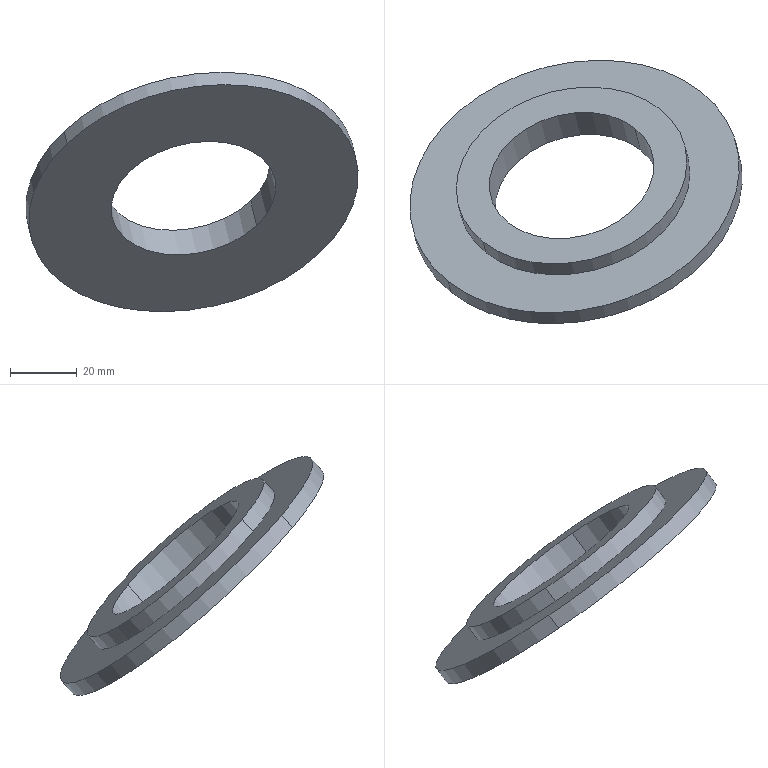Component | SolidWorks | FrictionWasher2-1 | 1 solid | 9 faces | box 99.33 x 78.81 x 71.5 mm | volume 38877 mm3 | cylinder 6 | plane 3 | commonest cylinder face diameters 70 x2 50 x2 100 x2 | material Copper
build123d program:
from build123d import *

# Parameters (mm, degrees)
SKETCH1_R           = 50
SKETCH1_R_2         = 35
BOSS_EXTRUDE1_DEPTH = 5
SKETCH1_3_R         = 35
SKETCH1_3_R_2       = 25
BOSS_EXTRUDE2_DEPTH = 10


with BuildPart() as part:
    # Sketch1 → Boss-Extrude1 (new body)
    with BuildSketch(Plane(origin=(0, 0, 0), x_dir=(1, 0, 0), z_dir=(0, 1, 0))):
        with Locations(Location((0, 0, 0), (0, 0, 270))):
            Circle(SKETCH1_R)
        with Locations(Location((0, 0, 0), (0, 0, 270))):
            Circle(SKETCH1_R_2, mode=Mode.SUBTRACT)
    extrude(amount=BOSS_EXTRUDE1_DEPTH)

    # Sketch1_3 → Boss-Extrude2 (add)
    with BuildSketch(Plane(origin=(0, 0, 0), x_dir=(1, 0, 0), z_dir=(0, 1, 0))):
        with Locations(Location((0, 0, 0), (0, 0, 270))):
            Circle(SKETCH1_3_R)
        with Locations(Location((0, 0, 0), (0, 0, 270))):
            Circle(SKETCH1_3_R_2, mode=Mode.SUBTRACT)
    extrude(amount=BOSS_EXTRUDE2_DEPTH)


solid = part.part

# Placed as in the assembly
solid = solid.moved(Location((-353.935, -1548.439, -88.002), (173.543, -77.716, 124.647)))
STEP:
#1=COLOUR_RGB('',0.7922,0.8196,0.9333);
#2=FILL_AREA_STYLE_COLOUR('',#1);
#3=FILL_AREA_STYLE('',(#2));
#4=SURFACE_STYLE_FILL_AREA(#3);
#5=SURFACE_SIDE_STYLE('',(#4));
#6=SURFACE_STYLE_USAGE(.BOTH.,#5);
#7=PRESENTATION_STYLE_ASSIGNMENT((#6));
#8=CARTESIAN_POINT('',(-12.963,-59.921,-3.626));
#9=VERTEX_POINT('',#8);
#10=CARTESIAN_POINT('',(-15.044,-61.487,-2.725));
#11=VERTEX_POINT('',#10);
#12=CARTESIAN_POINT('',(-14.003,-60.704,-3.175));
#13=DIRECTION('',(-0.175,0.6553,0.7348));
#14=DIRECTION('',(0.755,0.5683,-0.327));
#15=AXIS2_PLACEMENT_3D('',#12,#13,#14);
#16=CIRCLE('',#15,1.378);
#17=EDGE_CURVE('',#9,#11,#16,.T.);
#18=ORIENTED_EDGE('',*,*,#17,.F.);
#19=CARTESIAN_POINT('',(-12.928,-60.05,-3.771));
#20=VERTEX_POINT('',#19);
#21=CARTESIAN_POINT('',(-12.963,-59.921,-3.626));
#22=DIRECTION('',(0.175,-0.6553,-0.7348));
#23=VECTOR('',#22,39.37);
#24=LINE('',#21,#23);
#25=EDGE_CURVE('',#9,#20,#24,.T.);
#26=ORIENTED_EDGE('',*,*,#25,.T.);
#27=CARTESIAN_POINT('',(-15.009,-61.616,-2.869));
#28=VERTEX_POINT('',#27);
#29=CARTESIAN_POINT('',(-13.969,-60.833,-3.32));
#30=DIRECTION('',(-0.175,0.6553,0.7348));
#31=DIRECTION('',(0.755,0.5683,-0.327));
#32=AXIS2_PLACEMENT_3D('',#29,#30,#31);
#33=CIRCLE('',#32,1.378);
#34=EDGE_CURVE('',#20,#28,#33,.T.);
#35=ORIENTED_EDGE('',*,*,#34,.T.);
#36=CARTESIAN_POINT('',(-15.044,-61.487,-2.725));
#37=DIRECTION('',(0.175,-0.6553,-0.7348));
#38=VECTOR('',#37,39.37);
#39=LINE('',#36,#38);
#40=EDGE_CURVE('',#11,#28,#39,.T.);
#41=ORIENTED_EDGE('',*,*,#40,.F.);
#42=EDGE_LOOP('',(#18,#26,#35,#41));
#43=FACE_OUTER_BOUND('',#42,.T.);
#44=CARTESIAN_POINT('',(-14.003,-60.704,-3.175));
#45=DIRECTION('',(0.175,-0.6553,-0.7348));
#46=DIRECTION('',(-0.755,-0.5683,0.327));
#47=AXIS2_PLACEMENT_3D('',#44,#45,#46);
#48=CYLINDRICAL_SURFACE('',#47,1.378);
#49=ADVANCED_FACE('',(#43),#48,.T.);
#50=CARTESIAN_POINT('',(-14.747,-61.264,-2.854));
#51=VERTEX_POINT('',#50);
#52=CARTESIAN_POINT('',(-13.26,-60.145,-3.497));
#53=VERTEX_POINT('',#52);
#54=CARTESIAN_POINT('',(-14.003,-60.704,-3.175));
#55=DIRECTION('',(-0.175,0.6553,0.7348));
#56=DIRECTION('',(0.755,0.5683,-0.327));
#57=AXIS2_PLACEMENT_3D('',#54,#55,#56);
#58=CIRCLE('',#57,0.9843);
#59=EDGE_CURVE('',#51,#53,#58,.T.);
#60=ORIENTED_EDGE('',*,*,#59,.T.);
#61=CARTESIAN_POINT('',(-13.191,-60.403,-3.786));
#62=VERTEX_POINT('',#61);
#63=CARTESIAN_POINT('',(-13.26,-60.145,-3.497));
#64=DIRECTION('',(0.175,-0.6553,-0.7348));
#65=VECTOR('',#64,39.37);
#66=LINE('',#63,#65);
#67=EDGE_CURVE('',#53,#62,#66,.T.);
#68=ORIENTED_EDGE('',*,*,#67,.T.);
#69=CARTESIAN_POINT('',(-14.678,-61.522,-3.143));
#70=VERTEX_POINT('',#69);
#71=CARTESIAN_POINT('',(-13.934,-60.962,-3.465));
#72=DIRECTION('',(-0.175,0.6553,0.7348));
#73=DIRECTION('',(0.755,0.5683,-0.327));
#74=AXIS2_PLACEMENT_3D('',#71,#72,#73);
#75=CIRCLE('',#74,0.9843);
#76=EDGE_CURVE('',#70,#62,#75,.T.);
#77=ORIENTED_EDGE('',*,*,#76,.F.);
#78=CARTESIAN_POINT('',(-14.747,-61.264,-2.854));
#79=DIRECTION('',(0.175,-0.6553,-0.7348));
#80=VECTOR('',#79,39.37);
#81=LINE('',#78,#80);
#82=EDGE_CURVE('',#51,#70,#81,.T.);
#83=ORIENTED_EDGE('',*,*,#82,.F.);
#84=EDGE_LOOP('',(#60,#68,#77,#83));
#85=FACE_OUTER_BOUND('',#84,.T.);
#86=CARTESIAN_POINT('',(-14.003,-60.704,-3.175));
#87=DIRECTION('',(0.175,-0.6553,-0.7348));
#88=DIRECTION('',(-0.755,-0.5683,0.327));
#89=AXIS2_PLACEMENT_3D('',#86,#87,#88);
#90=CYLINDRICAL_SURFACE('',#89,0.9843);
#91=ADVANCED_FACE('',(#85),#90,.F.);
#92=CARTESIAN_POINT('',(-12.483,-59.714,-3.964));
#93=VERTEX_POINT('',#92);
#94=CARTESIAN_POINT('',(-15.455,-61.952,-2.676));
#95=VERTEX_POINT('',#94);
#96=CARTESIAN_POINT('',(-13.969,-60.833,-3.32));
#97=DIRECTION('',(-0.175,0.6553,0.7348));
#98=DIRECTION('',(0.755,0.5683,-0.327));
#99=AXIS2_PLACEMENT_3D('',#96,#97,#98);
#100=CIRCLE('',#99,1.969);
#101=EDGE_CURVE('',#93,#95,#100,.T.);
#102=ORIENTED_EDGE('',*,*,#101,.F.);
#103=CARTESIAN_POINT('',(-12.448,-59.843,-4.108));
#104=VERTEX_POINT('',#103);
#105=CARTESIAN_POINT('',(-12.483,-59.714,-3.964));
#106=DIRECTION('',(0.175,-0.6553,-0.7348));
#107=VECTOR('',#106,39.37);
#108=LINE('',#105,#107);
#109=EDGE_CURVE('',#93,#104,#108,.T.);
#110=ORIENTED_EDGE('',*,*,#109,.T.);
#111=CARTESIAN_POINT('',(-15.421,-62.081,-2.821));
#112=VERTEX_POINT('',#111);
#113=CARTESIAN_POINT('',(-13.934,-60.962,-3.465));
#114=DIRECTION('',(-0.175,0.6553,0.7348));
#115=DIRECTION('',(0.755,0.5683,-0.327));
#116=AXIS2_PLACEMENT_3D('',#113,#114,#115);
#117=CIRCLE('',#116,1.969);
#118=EDGE_CURVE('',#104,#112,#117,.T.);
#119=ORIENTED_EDGE('',*,*,#118,.T.);
#120=CARTESIAN_POINT('',(-15.455,-61.952,-2.676));
#121=DIRECTION('',(0.175,-0.6553,-0.7348));
#122=VECTOR('',#121,39.37);
#123=LINE('',#120,#122);
#124=EDGE_CURVE('',#95,#112,#123,.T.);
#125=ORIENTED_EDGE('',*,*,#124,.F.);
#126=EDGE_LOOP('',(#102,#110,#119,#125));
#127=FACE_OUTER_BOUND('',#126,.T.);
#128=CARTESIAN_POINT('',(-13.969,-60.833,-3.32));
#129=DIRECTION('',(0.175,-0.6553,-0.7348));
#130=DIRECTION('',(-0.755,-0.5683,0.327));
#131=AXIS2_PLACEMENT_3D('',#128,#129,#130);
#132=CYLINDRICAL_SURFACE('',#131,1.969);
#133=ADVANCED_FACE('',(#127),#132,.T.);
#134=ORIENTED_EDGE('',*,*,#109,.F.);
#135=CARTESIAN_POINT('',(-13.969,-60.833,-3.32));
#136=DIRECTION('',(-0.175,0.6553,0.7348));
#137=DIRECTION('',(0.755,0.5683,-0.327));
#138=AXIS2_PLACEMENT_3D('',#135,#136,#137);
#139=CIRCLE('',#138,1.969);
#140=EDGE_CURVE('',#95,#93,#139,.T.);
#141=ORIENTED_EDGE('',*,*,#140,.F.);
#142=ORIENTED_EDGE('',*,*,#124,.T.);
#143=CARTESIAN_POINT('',(-13.934,-60.962,-3.465));
#144=DIRECTION('',(-0.175,0.6553,0.7348));
#145=DIRECTION('',(0.755,0.5683,-0.327));
#146=AXIS2_PLACEMENT_3D('',#143,#144,#145);
#147=CIRCLE('',#146,1.969);
#148=EDGE_CURVE('',#112,#104,#147,.T.);
#149=ORIENTED_EDGE('',*,*,#148,.T.);
#150=EDGE_LOOP('',(#134,#141,#142,#149));
#151=FACE_OUTER_BOUND('',#150,.T.);
#152=CARTESIAN_POINT('',(-13.969,-60.833,-3.32));
#153=DIRECTION('',(0.175,-0.6553,-0.7348));
#154=DIRECTION('',(-0.755,-0.5683,0.327));
#155=AXIS2_PLACEMENT_3D('',#152,#153,#154);
#156=CYLINDRICAL_SURFACE('',#155,1.969);
#157=ADVANCED_FACE('',(#151),#156,.T.);
#158=CARTESIAN_POINT('',(-13.969,-60.833,-3.32));
#159=DIRECTION('',(-0.175,0.6553,0.7348));
#160=DIRECTION('',(0.755,0.5683,-0.327));
#161=AXIS2_PLACEMENT_3D('',#158,#159,#160);
#162=CIRCLE('',#161,1.378);
#163=EDGE_CURVE('',#28,#20,#162,.T.);
#164=ORIENTED_EDGE('',*,*,#163,.F.);
#165=ORIENTED_EDGE('',*,*,#34,.F.);
#166=EDGE_LOOP('',(#164,#165));
#167=FACE_BOUND('',#166,.T.);
#168=ORIENTED_EDGE('',*,*,#140,.T.);
#169=ORIENTED_EDGE('',*,*,#101,.T.);
#170=EDGE_LOOP('',(#168,#169));
#171=FACE_OUTER_BOUND('',#170,.T.);
#172=CARTESIAN_POINT('',(-13.969,-60.833,-3.32));
#173=DIRECTION('',(-0.175,0.6553,0.7348));
#174=DIRECTION('',(0.755,0.5683,-0.327));
#175=AXIS2_PLACEMENT_3D('',#172,#173,#174);
#176=PLANE('',#175);
#177=ADVANCED_FACE('',(#167,#171),#176,.T.);
#178=ORIENTED_EDGE('',*,*,#148,.F.);
#179=ORIENTED_EDGE('',*,*,#118,.F.);
#180=EDGE_LOOP('',(#178,#179));
#181=FACE_OUTER_BOUND('',#180,.T.);
#182=ORIENTED_EDGE('',*,*,#76,.T.);
#183=CARTESIAN_POINT('',(-13.934,-60.962,-3.465));
#184=DIRECTION('',(-0.175,0.6553,0.7348));
#185=DIRECTION('',(0.755,0.5683,-0.327));
#186=AXIS2_PLACEMENT_3D('',#183,#184,#185);
#187=CIRCLE('',#186,0.9843);
#188=EDGE_CURVE('',#62,#70,#187,.T.);
#189=ORIENTED_EDGE('',*,*,#188,.T.);
#190=EDGE_LOOP('',(#182,#189));
#191=FACE_BOUND('',#190,.T.);
#192=CARTESIAN_POINT('',(-13.934,-60.962,-3.465));
#193=DIRECTION('',(-0.175,0.6553,0.7348));
#194=DIRECTION('',(0.755,0.5683,-0.327));
#195=AXIS2_PLACEMENT_3D('',#192,#193,#194);
#196=PLANE('',#195);
#197=ADVANCED_FACE('',(#181,#191),#196,.F.);
#198=ORIENTED_EDGE('',*,*,#67,.F.);
#199=CARTESIAN_POINT('',(-14.003,-60.704,-3.175));
#200=DIRECTION('',(-0.175,0.6553,0.7348));
#201=DIRECTION('',(0.755,0.5683,-0.327));
#202=AXIS2_PLACEMENT_3D('',#199,#200,#201);
#203=CIRCLE('',#202,0.9843);
#204=EDGE_CURVE('',#53,#51,#203,.T.);
#205=ORIENTED_EDGE('',*,*,#204,.T.);
#206=ORIENTED_EDGE('',*,*,#82,.T.);
#207=ORIENTED_EDGE('',*,*,#188,.F.);
#208=EDGE_LOOP('',(#198,#205,#206,#207));
#209=FACE_OUTER_BOUND('',#208,.T.);
#210=CARTESIAN_POINT('',(-14.003,-60.704,-3.175));
#211=DIRECTION('',(0.175,-0.6553,-0.7348));
#212=DIRECTION('',(-0.755,-0.5683,0.327));
#213=AXIS2_PLACEMENT_3D('',#210,#211,#212);
#214=CYLINDRICAL_SURFACE('',#213,0.9843);
#215=ADVANCED_FACE('',(#209),#214,.F.);
#216=ORIENTED_EDGE('',*,*,#25,.F.);
#217=CARTESIAN_POINT('',(-14.003,-60.704,-3.175));
#218=DIRECTION('',(-0.175,0.6553,0.7348));
#219=DIRECTION('',(0.755,0.5683,-0.327));
#220=AXIS2_PLACEMENT_3D('',#217,#218,#219);
#221=CIRCLE('',#220,1.378);
#222=EDGE_CURVE('',#11,#9,#221,.T.);
#223=ORIENTED_EDGE('',*,*,#222,.F.);
#224=ORIENTED_EDGE('',*,*,#40,.T.);
#225=ORIENTED_EDGE('',*,*,#163,.T.);
#226=EDGE_LOOP('',(#216,#223,#224,#225));
#227=FACE_OUTER_BOUND('',#226,.T.);
#228=CARTESIAN_POINT('',(-14.003,-60.704,-3.175));
#229=DIRECTION('',(0.175,-0.6553,-0.7348));
#230=DIRECTION('',(-0.755,-0.5683,0.327));
#231=AXIS2_PLACEMENT_3D('',#228,#229,#230);
#232=CYLINDRICAL_SURFACE('',#231,1.378);
#233=ADVANCED_FACE('',(#227),#232,.T.);
#234=ORIENTED_EDGE('',*,*,#59,.F.);
#235=ORIENTED_EDGE('',*,*,#204,.F.);
#236=EDGE_LOOP('',(#234,#235));
#237=FACE_BOUND('',#236,.T.);
#238=ORIENTED_EDGE('',*,*,#222,.T.);
#239=ORIENTED_EDGE('',*,*,#17,.T.);
#240=EDGE_LOOP('',(#238,#239));
#241=FACE_OUTER_BOUND('',#240,.T.);
#242=CARTESIAN_POINT('',(-14.003,-60.704,-3.175));
#243=DIRECTION('',(-0.175,0.6553,0.7348));
#244=DIRECTION('',(0.755,0.5683,-0.327));
#245=AXIS2_PLACEMENT_3D('',#242,#243,#244);
#246=PLANE('',#245);
#247=ADVANCED_FACE('',(#237,#241),#246,.T.);
#248=CLOSED_SHELL('',(#49,#91,#133,#157,#177,#197,#215,#233,#247));
#249=MANIFOLD_SOLID_BREP('',#248);
#250=STYLED_ITEM('',(#7),#249);
#251=PRESENTATION_LAYER_ASSIGNMENT('','',(#250));
#252=CARTESIAN_POINT('',(0.,0.,0.));
#253=DIRECTION('',(0.,0.,1.));
#254=DIRECTION('',(1.,0.,0.));
#255=AXIS2_PLACEMENT_3D('',#252,#253,#254);
#256=(LENGTH_UNIT()NAMED_UNIT(*)SI_UNIT($,.METRE.));
#257=LENGTH_MEASURE_WITH_UNIT(LENGTH_MEASURE(0.0254),#256);
#258=DIMENSIONAL_EXPONENTS(1.,0.,0.,0.,0.,0.,0.);
#259=(CONVERSION_BASED_UNIT('',#257)LENGTH_UNIT()NAMED_UNIT(#258));
#260=UNCERTAINTY_MEASURE_WITH_UNIT(LENGTH_MEASURE(0.00001),#259,'','');
#261=(NAMED_UNIT(*)PLANE_ANGLE_UNIT()SI_UNIT($,.RADIAN.));
#262=(NAMED_UNIT(*)SI_UNIT($,.STERADIAN.)SOLID_ANGLE_UNIT());
#263=(GEOMETRIC_REPRESENTATION_CONTEXT(3)GLOBAL_UNCERTAINTY_ASSIGNED_CONTEXT((#260))GLOBAL_UNIT_ASSIGNED_CONTEXT((#259,#261,#262))REPRESENTATION_CONTEXT('',''));
#264=ADVANCED_BREP_SHAPE_REPRESENTATION('',(#249,#255),#263);
#265=(LENGTH_UNIT()NAMED_UNIT(*)SI_UNIT($,.METRE.));
#266=LENGTH_MEASURE_WITH_UNIT(LENGTH_MEASURE(0.0254),#265);
#267=DIMENSIONAL_EXPONENTS(1.,0.,0.,0.,0.,0.,0.);
#268=(CONVERSION_BASED_UNIT('',#266)LENGTH_UNIT()NAMED_UNIT(#267));
#269=UNCERTAINTY_MEASURE_WITH_UNIT(LENGTH_MEASURE(0.00001),#268,'','');
#270=(NAMED_UNIT(*)PLANE_ANGLE_UNIT()SI_UNIT($,.RADIAN.));
#271=(NAMED_UNIT(*)SI_UNIT($,.STERADIAN.)SOLID_ANGLE_UNIT());
#272=(GEOMETRIC_REPRESENTATION_CONTEXT(3)GLOBAL_UNCERTAINTY_ASSIGNED_CONTEXT((#269))GLOBAL_UNIT_ASSIGNED_CONTEXT((#268,#270,#271))REPRESENTATION_CONTEXT('',''));
#273=MECHANICAL_DESIGN_GEOMETRIC_PRESENTATION_REPRESENTATION('',(#250),#272);